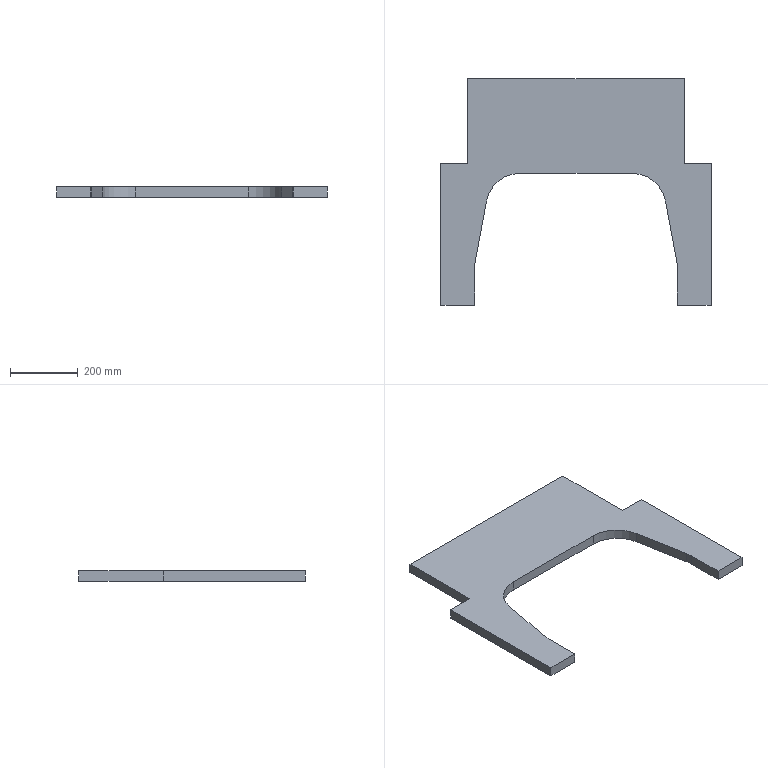Component | SolidWorks | JF21-80.1-1-3(_)-1-SOLID34-1 | 1 solid | 20 faces | box 800 x 670 x 30 mm | volume 8347939 mm3 | plane 16 | cylinder 4 | commonest cylinder face diameters 200 x4
STEP:
#1=COLOUR_RGB('',0.7922,0.8196,0.9333);
#2=FILL_AREA_STYLE_COLOUR('',#1);
#3=FILL_AREA_STYLE('',(#2));
#4=SURFACE_STYLE_FILL_AREA(#3);
#5=SURFACE_SIDE_STYLE('',(#4));
#6=SURFACE_STYLE_USAGE(.BOTH.,#5);
#7=PRESENTATION_STYLE_ASSIGNMENT((#6));
#8=CARTESIAN_POINT('',(15.748,-72.047,7.677));
#9=VERTEX_POINT('',#8);
#10=CARTESIAN_POINT('',(12.598,-72.047,7.677));
#11=VERTEX_POINT('',#10);
#12=CARTESIAN_POINT('',(12.598,-72.047,7.677));
#13=DIRECTION('',(-1.,0.,0.));
#14=VECTOR('',#13,39.37);
#15=LINE('',#12,#14);
#16=EDGE_CURVE('',#9,#11,#15,.T.);
#17=ORIENTED_EDGE('',*,*,#16,.T.);
#18=CARTESIAN_POINT('',(12.598,-72.047,8.858));
#19=VERTEX_POINT('',#18);
#20=CARTESIAN_POINT('',(12.598,-72.047,8.858));
#21=DIRECTION('',(0.,0.,-1.));
#22=VECTOR('',#21,39.37);
#23=LINE('',#20,#22);
#24=EDGE_CURVE('',#19,#11,#23,.T.);
#25=ORIENTED_EDGE('',*,*,#24,.F.);
#26=CARTESIAN_POINT('',(15.748,-72.047,8.858));
#27=VERTEX_POINT('',#26);
#28=CARTESIAN_POINT('',(12.598,-72.047,8.858));
#29=DIRECTION('',(-1.,0.,0.));
#30=VECTOR('',#29,39.37);
#31=LINE('',#28,#30);
#32=EDGE_CURVE('',#27,#19,#31,.T.);
#33=ORIENTED_EDGE('',*,*,#32,.F.);
#34=CARTESIAN_POINT('',(15.748,-72.047,8.858));
#35=DIRECTION('',(0.,0.,-1.));
#36=VECTOR('',#35,39.37);
#37=LINE('',#34,#36);
#38=EDGE_CURVE('',#27,#9,#37,.T.);
#39=ORIENTED_EDGE('',*,*,#38,.T.);
#40=EDGE_LOOP('',(#17,#25,#33,#39));
#41=FACE_OUTER_BOUND('',#40,.T.);
#42=CARTESIAN_POINT('',(12.598,-72.047,8.858));
#43=DIRECTION('',(0.,-1.,0.));
#44=DIRECTION('',(0.,0.,1.));
#45=AXIS2_PLACEMENT_3D('',#42,#43,#44);
#46=PLANE('',#45);
#47=ADVANCED_FACE('',(#41),#46,.F.);
#48=CARTESIAN_POINT('',(12.598,-62.205,7.677));
#49=VERTEX_POINT('',#48);
#50=CARTESIAN_POINT('',(12.598,-72.047,7.677));
#51=DIRECTION('',(0.,1.,0.));
#52=VECTOR('',#51,39.37);
#53=LINE('',#50,#52);
#54=EDGE_CURVE('',#11,#49,#53,.T.);
#55=ORIENTED_EDGE('',*,*,#54,.T.);
#56=CARTESIAN_POINT('',(12.598,-62.205,8.858));
#57=VERTEX_POINT('',#56);
#58=CARTESIAN_POINT('',(12.598,-62.205,8.858));
#59=DIRECTION('',(0.,0.,-1.));
#60=VECTOR('',#59,39.37);
#61=LINE('',#58,#60);
#62=EDGE_CURVE('',#57,#49,#61,.T.);
#63=ORIENTED_EDGE('',*,*,#62,.F.);
#64=CARTESIAN_POINT('',(12.598,-72.047,8.858));
#65=DIRECTION('',(0.,1.,0.));
#66=VECTOR('',#65,39.37);
#67=LINE('',#64,#66);
#68=EDGE_CURVE('',#19,#57,#67,.T.);
#69=ORIENTED_EDGE('',*,*,#68,.F.);
#70=ORIENTED_EDGE('',*,*,#24,.T.);
#71=EDGE_LOOP('',(#55,#63,#69,#70));
#72=FACE_OUTER_BOUND('',#71,.T.);
#73=CARTESIAN_POINT('',(12.598,-72.047,8.858));
#74=DIRECTION('',(-1.,0.,0.));
#75=DIRECTION('',(0.,0.,-1.));
#76=AXIS2_PLACEMENT_3D('',#73,#74,#75);
#77=PLANE('',#76);
#78=ADVANCED_FACE('',(#72),#77,.F.);
#79=CARTESIAN_POINT('',(-12.598,-62.205,7.677));
#80=VERTEX_POINT('',#79);
#81=CARTESIAN_POINT('',(-12.598,-62.205,7.677));
#82=DIRECTION('',(-1.,0.,0.));
#83=VECTOR('',#82,39.37);
#84=LINE('',#81,#83);
#85=EDGE_CURVE('',#49,#80,#84,.T.);
#86=ORIENTED_EDGE('',*,*,#85,.T.);
#87=CARTESIAN_POINT('',(-12.598,-62.205,8.858));
#88=VERTEX_POINT('',#87);
#89=CARTESIAN_POINT('',(-12.598,-62.205,8.858));
#90=DIRECTION('',(0.,0.,-1.));
#91=VECTOR('',#90,39.37);
#92=LINE('',#89,#91);
#93=EDGE_CURVE('',#88,#80,#92,.T.);
#94=ORIENTED_EDGE('',*,*,#93,.F.);
#95=CARTESIAN_POINT('',(-12.598,-62.205,8.858));
#96=DIRECTION('',(-1.,0.,0.));
#97=VECTOR('',#96,39.37);
#98=LINE('',#95,#97);
#99=EDGE_CURVE('',#57,#88,#98,.T.);
#100=ORIENTED_EDGE('',*,*,#99,.F.);
#101=ORIENTED_EDGE('',*,*,#62,.T.);
#102=EDGE_LOOP('',(#86,#94,#100,#101));
#103=FACE_OUTER_BOUND('',#102,.T.);
#104=CARTESIAN_POINT('',(-12.598,-62.205,8.858));
#105=DIRECTION('',(0.,-1.,0.));
#106=DIRECTION('',(0.,0.,1.));
#107=AXIS2_PLACEMENT_3D('',#104,#105,#106);
#108=PLANE('',#107);
#109=ADVANCED_FACE('',(#103),#108,.F.);
#110=CARTESIAN_POINT('',(-12.598,-72.047,7.677));
#111=VERTEX_POINT('',#110);
#112=CARTESIAN_POINT('',(-12.598,-72.047,7.677));
#113=DIRECTION('',(0.,-1.,0.));
#114=VECTOR('',#113,39.37);
#115=LINE('',#112,#114);
#116=EDGE_CURVE('',#80,#111,#115,.T.);
#117=ORIENTED_EDGE('',*,*,#116,.T.);
#118=CARTESIAN_POINT('',(-12.598,-72.047,8.858));
#119=VERTEX_POINT('',#118);
#120=CARTESIAN_POINT('',(-12.598,-72.047,8.858));
#121=DIRECTION('',(0.,0.,-1.));
#122=VECTOR('',#121,39.37);
#123=LINE('',#120,#122);
#124=EDGE_CURVE('',#119,#111,#123,.T.);
#125=ORIENTED_EDGE('',*,*,#124,.F.);
#126=CARTESIAN_POINT('',(-12.598,-72.047,8.858));
#127=DIRECTION('',(0.,-1.,0.));
#128=VECTOR('',#127,39.37);
#129=LINE('',#126,#128);
#130=EDGE_CURVE('',#88,#119,#129,.T.);
#131=ORIENTED_EDGE('',*,*,#130,.F.);
#132=ORIENTED_EDGE('',*,*,#93,.T.);
#133=EDGE_LOOP('',(#117,#125,#131,#132));
#134=FACE_OUTER_BOUND('',#133,.T.);
#135=CARTESIAN_POINT('',(-12.598,-72.047,8.858));
#136=DIRECTION('',(1.,0.,0.));
#137=DIRECTION('',(0.,0.,1.));
#138=AXIS2_PLACEMENT_3D('',#135,#136,#137);
#139=PLANE('',#138);
#140=ADVANCED_FACE('',(#134),#139,.F.);
#141=CARTESIAN_POINT('',(-15.748,-72.047,7.677));
#142=VERTEX_POINT('',#141);
#143=CARTESIAN_POINT('',(-12.598,-72.047,7.677));
#144=DIRECTION('',(-1.,0.,0.));
#145=VECTOR('',#144,39.37);
#146=LINE('',#143,#145);
#147=EDGE_CURVE('',#111,#142,#146,.T.);
#148=ORIENTED_EDGE('',*,*,#147,.T.);
#149=CARTESIAN_POINT('',(-15.748,-72.047,8.858));
#150=VERTEX_POINT('',#149);
#151=CARTESIAN_POINT('',(-15.748,-72.047,8.858));
#152=DIRECTION('',(0.,0.,-1.));
#153=VECTOR('',#152,39.37);
#154=LINE('',#151,#153);
#155=EDGE_CURVE('',#150,#142,#154,.T.);
#156=ORIENTED_EDGE('',*,*,#155,.F.);
#157=CARTESIAN_POINT('',(-12.598,-72.047,8.858));
#158=DIRECTION('',(-1.,0.,0.));
#159=VECTOR('',#158,39.37);
#160=LINE('',#157,#159);
#161=EDGE_CURVE('',#119,#150,#160,.T.);
#162=ORIENTED_EDGE('',*,*,#161,.F.);
#163=ORIENTED_EDGE('',*,*,#124,.T.);
#164=EDGE_LOOP('',(#148,#156,#162,#163));
#165=FACE_OUTER_BOUND('',#164,.T.);
#166=CARTESIAN_POINT('',(-12.598,-72.047,8.858));
#167=DIRECTION('',(0.,-1.,0.));
#168=DIRECTION('',(0.,0.,1.));
#169=AXIS2_PLACEMENT_3D('',#166,#167,#168);
#170=PLANE('',#169);
#171=ADVANCED_FACE('',(#165),#170,.F.);
#172=CARTESIAN_POINT('',(-15.748,-88.583,7.677));
#173=VERTEX_POINT('',#172);
#174=CARTESIAN_POINT('',(-15.748,-72.047,7.677));
#175=DIRECTION('',(0.,-1.,0.));
#176=VECTOR('',#175,39.37);
#177=LINE('',#174,#176);
#178=EDGE_CURVE('',#142,#173,#177,.T.);
#179=ORIENTED_EDGE('',*,*,#178,.T.);
#180=CARTESIAN_POINT('',(-15.748,-88.583,8.858));
#181=VERTEX_POINT('',#180);
#182=CARTESIAN_POINT('',(-15.748,-88.583,8.858));
#183=DIRECTION('',(0.,0.,-1.));
#184=VECTOR('',#183,39.37);
#185=LINE('',#182,#184);
#186=EDGE_CURVE('',#181,#173,#185,.T.);
#187=ORIENTED_EDGE('',*,*,#186,.F.);
#188=CARTESIAN_POINT('',(-15.748,-72.047,8.858));
#189=DIRECTION('',(0.,-1.,0.));
#190=VECTOR('',#189,39.37);
#191=LINE('',#188,#190);
#192=EDGE_CURVE('',#150,#181,#191,.T.);
#193=ORIENTED_EDGE('',*,*,#192,.F.);
#194=ORIENTED_EDGE('',*,*,#155,.T.);
#195=EDGE_LOOP('',(#179,#187,#193,#194));
#196=FACE_OUTER_BOUND('',#195,.T.);
#197=CARTESIAN_POINT('',(-15.748,-72.047,8.858));
#198=DIRECTION('',(1.,0.,0.));
#199=DIRECTION('',(0.,0.,1.));
#200=AXIS2_PLACEMENT_3D('',#197,#198,#199);
#201=PLANE('',#200);
#202=ADVANCED_FACE('',(#196),#201,.F.);
#203=CARTESIAN_POINT('',(-11.811,-88.583,7.677));
#204=VERTEX_POINT('',#203);
#205=CARTESIAN_POINT('',(-11.811,-88.583,7.677));
#206=DIRECTION('',(1.,0.,0.));
#207=VECTOR('',#206,39.37);
#208=LINE('',#205,#207);
#209=EDGE_CURVE('',#173,#204,#208,.T.);
#210=ORIENTED_EDGE('',*,*,#209,.T.);
#211=CARTESIAN_POINT('',(-11.811,-88.583,8.858));
#212=VERTEX_POINT('',#211);
#213=CARTESIAN_POINT('',(-11.811,-88.583,8.858));
#214=DIRECTION('',(0.,0.,-1.));
#215=VECTOR('',#214,39.37);
#216=LINE('',#213,#215);
#217=EDGE_CURVE('',#212,#204,#216,.T.);
#218=ORIENTED_EDGE('',*,*,#217,.F.);
#219=CARTESIAN_POINT('',(-11.811,-88.583,8.858));
#220=DIRECTION('',(1.,0.,0.));
#221=VECTOR('',#220,39.37);
#222=LINE('',#219,#221);
#223=EDGE_CURVE('',#181,#212,#222,.T.);
#224=ORIENTED_EDGE('',*,*,#223,.F.);
#225=ORIENTED_EDGE('',*,*,#186,.T.);
#226=EDGE_LOOP('',(#210,#218,#224,#225));
#227=FACE_OUTER_BOUND('',#226,.T.);
#228=CARTESIAN_POINT('',(-11.811,-88.583,8.858));
#229=DIRECTION('',(0.,1.,0.));
#230=DIRECTION('',(0.,0.,-1.));
#231=AXIS2_PLACEMENT_3D('',#228,#229,#230);
#232=PLANE('',#231);
#233=ADVANCED_FACE('',(#227),#232,.F.);
#234=CARTESIAN_POINT('',(-11.811,-84.22,7.677));
#235=VERTEX_POINT('',#234);
#236=CARTESIAN_POINT('',(-11.811,-84.22,7.677));
#237=DIRECTION('',(0.,1.,0.));
#238=VECTOR('',#237,39.37);
#239=LINE('',#236,#238);
#240=EDGE_CURVE('',#204,#235,#239,.T.);
#241=ORIENTED_EDGE('',*,*,#240,.T.);
#242=CARTESIAN_POINT('',(-11.811,-84.22,8.858));
#243=VERTEX_POINT('',#242);
#244=CARTESIAN_POINT('',(-11.811,-84.22,8.858));
#245=DIRECTION('',(0.,0.,-1.));
#246=VECTOR('',#245,39.37);
#247=LINE('',#244,#246);
#248=EDGE_CURVE('',#243,#235,#247,.T.);
#249=ORIENTED_EDGE('',*,*,#248,.F.);
#250=CARTESIAN_POINT('',(-11.811,-84.22,8.858));
#251=DIRECTION('',(0.,1.,0.));
#252=VECTOR('',#251,39.37);
#253=LINE('',#250,#252);
#254=EDGE_CURVE('',#212,#243,#253,.T.);
#255=ORIENTED_EDGE('',*,*,#254,.F.);
#256=ORIENTED_EDGE('',*,*,#217,.T.);
#257=EDGE_LOOP('',(#241,#249,#255,#256));
#258=FACE_OUTER_BOUND('',#257,.T.);
#259=CARTESIAN_POINT('',(-11.811,-84.22,8.858));
#260=DIRECTION('',(-1.,0.,0.));
#261=DIRECTION('',(0.,0.,-1.));
#262=AXIS2_PLACEMENT_3D('',#259,#260,#261);
#263=PLANE('',#262);
#264=ADVANCED_FACE('',(#258),#263,.F.);
#265=CARTESIAN_POINT('',(-11.745,-83.503,7.677));
#266=VERTEX_POINT('',#265);
#267=CARTESIAN_POINT('',(-7.874,-84.22,7.677));
#268=DIRECTION('',(0.,0.,-1.));
#269=DIRECTION('',(1.,0.,0.));
#270=AXIS2_PLACEMENT_3D('',#267,#268,#269);
#271=CIRCLE('',#270,3.937);
#272=EDGE_CURVE('',#235,#266,#271,.T.);
#273=ORIENTED_EDGE('',*,*,#272,.T.);
#274=CARTESIAN_POINT('',(-11.745,-83.503,8.858));
#275=VERTEX_POINT('',#274);
#276=CARTESIAN_POINT('',(-11.745,-83.503,8.858));
#277=DIRECTION('',(0.,0.,-1.));
#278=VECTOR('',#277,39.37);
#279=LINE('',#276,#278);
#280=EDGE_CURVE('',#275,#266,#279,.T.);
#281=ORIENTED_EDGE('',*,*,#280,.F.);
#282=CARTESIAN_POINT('',(-7.874,-84.22,8.858));
#283=DIRECTION('',(0.,0.,-1.));
#284=DIRECTION('',(1.,0.,0.));
#285=AXIS2_PLACEMENT_3D('',#282,#283,#284);
#286=CIRCLE('',#285,3.937);
#287=EDGE_CURVE('',#243,#275,#286,.T.);
#288=ORIENTED_EDGE('',*,*,#287,.F.);
#289=ORIENTED_EDGE('',*,*,#248,.T.);
#290=EDGE_LOOP('',(#273,#281,#288,#289));
#291=FACE_OUTER_BOUND('',#290,.T.);
#292=CARTESIAN_POINT('',(-7.874,-84.22,8.858));
#293=DIRECTION('',(0.,0.,-1.));
#294=DIRECTION('',(1.,0.,0.));
#295=AXIS2_PLACEMENT_3D('',#292,#293,#294);
#296=CYLINDRICAL_SURFACE('',#295,3.937);
#297=ADVANCED_FACE('',(#291),#296,.F.);
#298=CARTESIAN_POINT('',(-10.439,-76.448,7.677));
#299=VERTEX_POINT('',#298);
#300=CARTESIAN_POINT('',(-10.439,-76.448,7.677));
#301=DIRECTION('',(0.1821,0.9833,0.));
#302=VECTOR('',#301,39.37);
#303=LINE('',#300,#302);
#304=EDGE_CURVE('',#266,#299,#303,.T.);
#305=ORIENTED_EDGE('',*,*,#304,.T.);
#306=CARTESIAN_POINT('',(-10.439,-76.448,8.858));
#307=VERTEX_POINT('',#306);
#308=CARTESIAN_POINT('',(-10.439,-76.448,8.858));
#309=DIRECTION('',(0.,0.,-1.));
#310=VECTOR('',#309,39.37);
#311=LINE('',#308,#310);
#312=EDGE_CURVE('',#307,#299,#311,.T.);
#313=ORIENTED_EDGE('',*,*,#312,.F.);
#314=CARTESIAN_POINT('',(-10.439,-76.448,8.858));
#315=DIRECTION('',(0.1821,0.9833,0.));
#316=VECTOR('',#315,39.37);
#317=LINE('',#314,#316);
#318=EDGE_CURVE('',#275,#307,#317,.T.);
#319=ORIENTED_EDGE('',*,*,#318,.F.);
#320=ORIENTED_EDGE('',*,*,#280,.T.);
#321=EDGE_LOOP('',(#305,#313,#319,#320));
#322=FACE_OUTER_BOUND('',#321,.T.);
#323=CARTESIAN_POINT('',(-10.439,-76.448,8.858));
#324=DIRECTION('',(-0.9833,0.1821,0.));
#325=DIRECTION('',(0.1821,0.9833,0.));
#326=AXIS2_PLACEMENT_3D('',#323,#324,#325);
#327=PLANE('',#326);
#328=ADVANCED_FACE('',(#322),#327,.F.);
#329=CARTESIAN_POINT('',(-6.568,-73.228,7.677));
#330=VERTEX_POINT('',#329);
#331=CARTESIAN_POINT('',(-6.568,-77.165,7.677));
#332=DIRECTION('',(0.,0.,-1.));
#333=DIRECTION('',(1.,0.,0.));
#334=AXIS2_PLACEMENT_3D('',#331,#332,#333);
#335=CIRCLE('',#334,3.937);
#336=EDGE_CURVE('',#299,#330,#335,.T.);
#337=ORIENTED_EDGE('',*,*,#336,.T.);
#338=CARTESIAN_POINT('',(-6.568,-73.228,8.858));
#339=VERTEX_POINT('',#338);
#340=CARTESIAN_POINT('',(-6.568,-73.228,8.858));
#341=DIRECTION('',(0.,0.,-1.));
#342=VECTOR('',#341,39.37);
#343=LINE('',#340,#342);
#344=EDGE_CURVE('',#339,#330,#343,.T.);
#345=ORIENTED_EDGE('',*,*,#344,.F.);
#346=CARTESIAN_POINT('',(-6.568,-77.165,8.858));
#347=DIRECTION('',(0.,0.,-1.));
#348=DIRECTION('',(1.,0.,0.));
#349=AXIS2_PLACEMENT_3D('',#346,#347,#348);
#350=CIRCLE('',#349,3.937);
#351=EDGE_CURVE('',#307,#339,#350,.T.);
#352=ORIENTED_EDGE('',*,*,#351,.F.);
#353=ORIENTED_EDGE('',*,*,#312,.T.);
#354=EDGE_LOOP('',(#337,#345,#352,#353));
#355=FACE_OUTER_BOUND('',#354,.T.);
#356=CARTESIAN_POINT('',(-6.568,-77.165,8.858));
#357=DIRECTION('',(0.,0.,-1.));
#358=DIRECTION('',(1.,0.,0.));
#359=AXIS2_PLACEMENT_3D('',#356,#357,#358);
#360=CYLINDRICAL_SURFACE('',#359,3.937);
#361=ADVANCED_FACE('',(#355),#360,.F.);
#362=CARTESIAN_POINT('',(6.568,-73.228,7.677));
#363=VERTEX_POINT('',#362);
#364=CARTESIAN_POINT('',(6.568,-73.228,7.677));
#365=DIRECTION('',(1.,0.,0.));
#366=VECTOR('',#365,39.37);
#367=LINE('',#364,#366);
#368=EDGE_CURVE('',#330,#363,#367,.T.);
#369=ORIENTED_EDGE('',*,*,#368,.T.);
#370=CARTESIAN_POINT('',(6.568,-73.228,8.858));
#371=VERTEX_POINT('',#370);
#372=CARTESIAN_POINT('',(6.568,-73.228,8.858));
#373=DIRECTION('',(0.,0.,-1.));
#374=VECTOR('',#373,39.37);
#375=LINE('',#372,#374);
#376=EDGE_CURVE('',#371,#363,#375,.T.);
#377=ORIENTED_EDGE('',*,*,#376,.F.);
#378=CARTESIAN_POINT('',(6.568,-73.228,8.858));
#379=DIRECTION('',(1.,0.,0.));
#380=VECTOR('',#379,39.37);
#381=LINE('',#378,#380);
#382=EDGE_CURVE('',#339,#371,#381,.T.);
#383=ORIENTED_EDGE('',*,*,#382,.F.);
#384=ORIENTED_EDGE('',*,*,#344,.T.);
#385=EDGE_LOOP('',(#369,#377,#383,#384));
#386=FACE_OUTER_BOUND('',#385,.T.);
#387=CARTESIAN_POINT('',(6.568,-73.228,8.858));
#388=DIRECTION('',(0.,1.,0.));
#389=DIRECTION('',(0.,0.,-1.));
#390=AXIS2_PLACEMENT_3D('',#387,#388,#389);
#391=PLANE('',#390);
#392=ADVANCED_FACE('',(#386),#391,.F.);
#393=CARTESIAN_POINT('',(10.439,-76.448,7.677));
#394=VERTEX_POINT('',#393);
#395=CARTESIAN_POINT('',(6.568,-77.165,7.677));
#396=DIRECTION('',(0.,0.,-1.));
#397=DIRECTION('',(1.,0.,0.));
#398=AXIS2_PLACEMENT_3D('',#395,#396,#397);
#399=CIRCLE('',#398,3.937);
#400=EDGE_CURVE('',#363,#394,#399,.T.);
#401=ORIENTED_EDGE('',*,*,#400,.T.);
#402=CARTESIAN_POINT('',(10.439,-76.448,8.858));
#403=VERTEX_POINT('',#402);
#404=CARTESIAN_POINT('',(10.439,-76.448,8.858));
#405=DIRECTION('',(0.,0.,-1.));
#406=VECTOR('',#405,39.37);
#407=LINE('',#404,#406);
#408=EDGE_CURVE('',#403,#394,#407,.T.);
#409=ORIENTED_EDGE('',*,*,#408,.F.);
#410=CARTESIAN_POINT('',(6.568,-77.165,8.858));
#411=DIRECTION('',(0.,0.,-1.));
#412=DIRECTION('',(1.,0.,0.));
#413=AXIS2_PLACEMENT_3D('',#410,#411,#412);
#414=CIRCLE('',#413,3.937);
#415=EDGE_CURVE('',#371,#403,#414,.T.);
#416=ORIENTED_EDGE('',*,*,#415,.F.);
#417=ORIENTED_EDGE('',*,*,#376,.T.);
#418=EDGE_LOOP('',(#401,#409,#416,#417));
#419=FACE_OUTER_BOUND('',#418,.T.);
#420=CARTESIAN_POINT('',(6.568,-77.165,8.858));
#421=DIRECTION('',(0.,0.,-1.));
#422=DIRECTION('',(1.,0.,0.));
#423=AXIS2_PLACEMENT_3D('',#420,#421,#422);
#424=CYLINDRICAL_SURFACE('',#423,3.937);
#425=ADVANCED_FACE('',(#419),#424,.F.);
#426=CARTESIAN_POINT('',(11.745,-83.503,7.677));
#427=VERTEX_POINT('',#426);
#428=CARTESIAN_POINT('',(11.745,-83.503,7.677));
#429=DIRECTION('',(0.1821,-0.9833,0.));
#430=VECTOR('',#429,39.37);
#431=LINE('',#428,#430);
#432=EDGE_CURVE('',#394,#427,#431,.T.);
#433=ORIENTED_EDGE('',*,*,#432,.T.);
#434=CARTESIAN_POINT('',(11.745,-83.503,8.858));
#435=VERTEX_POINT('',#434);
#436=CARTESIAN_POINT('',(11.745,-83.503,8.858));
#437=DIRECTION('',(0.,0.,-1.));
#438=VECTOR('',#437,39.37);
#439=LINE('',#436,#438);
#440=EDGE_CURVE('',#435,#427,#439,.T.);
#441=ORIENTED_EDGE('',*,*,#440,.F.);
#442=CARTESIAN_POINT('',(11.745,-83.503,8.858));
#443=DIRECTION('',(0.1821,-0.9833,0.));
#444=VECTOR('',#443,39.37);
#445=LINE('',#442,#444);
#446=EDGE_CURVE('',#403,#435,#445,.T.);
#447=ORIENTED_EDGE('',*,*,#446,.F.);
#448=ORIENTED_EDGE('',*,*,#408,.T.);
#449=EDGE_LOOP('',(#433,#441,#447,#448));
#450=FACE_OUTER_BOUND('',#449,.T.);
#451=CARTESIAN_POINT('',(11.745,-83.503,8.858));
#452=DIRECTION('',(0.9833,0.1821,0.));
#453=DIRECTION('',(0.1821,-0.9833,0.));
#454=AXIS2_PLACEMENT_3D('',#451,#452,#453);
#455=PLANE('',#454);
#456=ADVANCED_FACE('',(#450),#455,.F.);
#457=CARTESIAN_POINT('',(11.811,-84.22,7.677));
#458=VERTEX_POINT('',#457);
#459=CARTESIAN_POINT('',(7.874,-84.22,7.677));
#460=DIRECTION('',(0.,0.,-1.));
#461=DIRECTION('',(1.,0.,0.));
#462=AXIS2_PLACEMENT_3D('',#459,#460,#461);
#463=CIRCLE('',#462,3.937);
#464=EDGE_CURVE('',#427,#458,#463,.T.);
#465=ORIENTED_EDGE('',*,*,#464,.T.);
#466=CARTESIAN_POINT('',(11.811,-84.22,8.858));
#467=VERTEX_POINT('',#466);
#468=CARTESIAN_POINT('',(11.811,-84.22,8.858));
#469=DIRECTION('',(0.,0.,-1.));
#470=VECTOR('',#469,39.37);
#471=LINE('',#468,#470);
#472=EDGE_CURVE('',#467,#458,#471,.T.);
#473=ORIENTED_EDGE('',*,*,#472,.F.);
#474=CARTESIAN_POINT('',(7.874,-84.22,8.858));
#475=DIRECTION('',(0.,0.,-1.));
#476=DIRECTION('',(1.,0.,0.));
#477=AXIS2_PLACEMENT_3D('',#474,#475,#476);
#478=CIRCLE('',#477,3.937);
#479=EDGE_CURVE('',#435,#467,#478,.T.);
#480=ORIENTED_EDGE('',*,*,#479,.F.);
#481=ORIENTED_EDGE('',*,*,#440,.T.);
#482=EDGE_LOOP('',(#465,#473,#480,#481));
#483=FACE_OUTER_BOUND('',#482,.T.);
#484=CARTESIAN_POINT('',(7.874,-84.22,8.858));
#485=DIRECTION('',(0.,0.,-1.));
#486=DIRECTION('',(1.,0.,0.));
#487=AXIS2_PLACEMENT_3D('',#484,#485,#486);
#488=CYLINDRICAL_SURFACE('',#487,3.937);
#489=ADVANCED_FACE('',(#483),#488,.F.);
#490=CARTESIAN_POINT('',(11.811,-88.583,7.677));
#491=VERTEX_POINT('',#490);
#492=CARTESIAN_POINT('',(11.811,-88.583,7.677));
#493=DIRECTION('',(-0.,-1.,0.));
#494=VECTOR('',#493,39.37);
#495=LINE('',#492,#494);
#496=EDGE_CURVE('',#458,#491,#495,.T.);
#497=ORIENTED_EDGE('',*,*,#496,.T.);
#498=CARTESIAN_POINT('',(11.811,-88.583,8.858));
#499=VERTEX_POINT('',#498);
#500=CARTESIAN_POINT('',(11.811,-88.583,8.858));
#501=DIRECTION('',(0.,0.,-1.));
#502=VECTOR('',#501,39.37);
#503=LINE('',#500,#502);
#504=EDGE_CURVE('',#499,#491,#503,.T.);
#505=ORIENTED_EDGE('',*,*,#504,.F.);
#506=CARTESIAN_POINT('',(11.811,-88.583,8.858));
#507=DIRECTION('',(-0.,-1.,0.));
#508=VECTOR('',#507,39.37);
#509=LINE('',#506,#508);
#510=EDGE_CURVE('',#467,#499,#509,.T.);
#511=ORIENTED_EDGE('',*,*,#510,.F.);
#512=ORIENTED_EDGE('',*,*,#472,.T.);
#513=EDGE_LOOP('',(#497,#505,#511,#512));
#514=FACE_OUTER_BOUND('',#513,.T.);
#515=CARTESIAN_POINT('',(11.811,-88.583,8.858));
#516=DIRECTION('',(1.,-0.,0.));
#517=DIRECTION('',(-0.,-1.,0.));
#518=AXIS2_PLACEMENT_3D('',#515,#516,#517);
#519=PLANE('',#518);
#520=ADVANCED_FACE('',(#514),#519,.F.);
#521=CARTESIAN_POINT('',(15.748,-88.583,7.677));
#522=VERTEX_POINT('',#521);
#523=CARTESIAN_POINT('',(15.748,-88.583,7.677));
#524=DIRECTION('',(1.,0.,0.));
#525=VECTOR('',#524,39.37);
#526=LINE('',#523,#525);
#527=EDGE_CURVE('',#491,#522,#526,.T.);
#528=ORIENTED_EDGE('',*,*,#527,.T.);
#529=CARTESIAN_POINT('',(15.748,-88.583,8.858));
#530=VERTEX_POINT('',#529);
#531=CARTESIAN_POINT('',(15.748,-88.583,8.858));
#532=DIRECTION('',(0.,0.,-1.));
#533=VECTOR('',#532,39.37);
#534=LINE('',#531,#533);
#535=EDGE_CURVE('',#530,#522,#534,.T.);
#536=ORIENTED_EDGE('',*,*,#535,.F.);
#537=CARTESIAN_POINT('',(15.748,-88.583,8.858));
#538=DIRECTION('',(1.,0.,0.));
#539=VECTOR('',#538,39.37);
#540=LINE('',#537,#539);
#541=EDGE_CURVE('',#499,#530,#540,.T.);
#542=ORIENTED_EDGE('',*,*,#541,.F.);
#543=ORIENTED_EDGE('',*,*,#504,.T.);
#544=EDGE_LOOP('',(#528,#536,#542,#543));
#545=FACE_OUTER_BOUND('',#544,.T.);
#546=CARTESIAN_POINT('',(15.748,-88.583,8.858));
#547=DIRECTION('',(0.,1.,0.));
#548=DIRECTION('',(0.,0.,-1.));
#549=AXIS2_PLACEMENT_3D('',#546,#547,#548);
#550=PLANE('',#549);
#551=ADVANCED_FACE('',(#545),#550,.F.);
#552=CARTESIAN_POINT('',(15.748,-72.047,7.677));
#553=DIRECTION('',(0.,1.,0.));
#554=VECTOR('',#553,39.37);
#555=LINE('',#552,#554);
#556=EDGE_CURVE('',#522,#9,#555,.T.);
#557=ORIENTED_EDGE('',*,*,#556,.T.);
#558=ORIENTED_EDGE('',*,*,#38,.F.);
#559=CARTESIAN_POINT('',(15.748,-72.047,8.858));
#560=DIRECTION('',(0.,1.,0.));
#561=VECTOR('',#560,39.37);
#562=LINE('',#559,#561);
#563=EDGE_CURVE('',#530,#27,#562,.T.);
#564=ORIENTED_EDGE('',*,*,#563,.F.);
#565=ORIENTED_EDGE('',*,*,#535,.T.);
#566=EDGE_LOOP('',(#557,#558,#564,#565));
#567=FACE_OUTER_BOUND('',#566,.T.);
#568=CARTESIAN_POINT('',(15.748,-72.047,8.858));
#569=DIRECTION('',(-1.,0.,0.));
#570=DIRECTION('',(0.,0.,-1.));
#571=AXIS2_PLACEMENT_3D('',#568,#569,#570);
#572=PLANE('',#571);
#573=ADVANCED_FACE('',(#567),#572,.F.);
#574=ORIENTED_EDGE('',*,*,#32,.T.);
#575=ORIENTED_EDGE('',*,*,#68,.T.);
#576=ORIENTED_EDGE('',*,*,#99,.T.);
#577=ORIENTED_EDGE('',*,*,#130,.T.);
#578=ORIENTED_EDGE('',*,*,#161,.T.);
#579=ORIENTED_EDGE('',*,*,#192,.T.);
#580=ORIENTED_EDGE('',*,*,#223,.T.);
#581=ORIENTED_EDGE('',*,*,#254,.T.);
#582=ORIENTED_EDGE('',*,*,#287,.T.);
#583=ORIENTED_EDGE('',*,*,#318,.T.);
#584=ORIENTED_EDGE('',*,*,#351,.T.);
#585=ORIENTED_EDGE('',*,*,#382,.T.);
#586=ORIENTED_EDGE('',*,*,#415,.T.);
#587=ORIENTED_EDGE('',*,*,#446,.T.);
#588=ORIENTED_EDGE('',*,*,#479,.T.);
#589=ORIENTED_EDGE('',*,*,#510,.T.);
#590=ORIENTED_EDGE('',*,*,#541,.T.);
#591=ORIENTED_EDGE('',*,*,#563,.T.);
#592=EDGE_LOOP('',(#574,#575,#576,#577,#578,#579,#580,#581,#582,#583,#584,#585,#586,#587,#588,#589,#590,#591));
#593=FACE_OUTER_BOUND('',#592,.T.);
#594=CARTESIAN_POINT('',(7.874,-84.22,8.858));
#595=DIRECTION('',(0.,0.,1.));
#596=DIRECTION('',(-1.,0.,0.));
#597=AXIS2_PLACEMENT_3D('',#594,#595,#596);
#598=PLANE('',#597);
#599=ADVANCED_FACE('',(#593),#598,.T.);
#600=ORIENTED_EDGE('',*,*,#16,.F.);
#601=ORIENTED_EDGE('',*,*,#556,.F.);
#602=ORIENTED_EDGE('',*,*,#527,.F.);
#603=ORIENTED_EDGE('',*,*,#496,.F.);
#604=ORIENTED_EDGE('',*,*,#464,.F.);
#605=ORIENTED_EDGE('',*,*,#432,.F.);
#606=ORIENTED_EDGE('',*,*,#400,.F.);
#607=ORIENTED_EDGE('',*,*,#368,.F.);
#608=ORIENTED_EDGE('',*,*,#336,.F.);
#609=ORIENTED_EDGE('',*,*,#304,.F.);
#610=ORIENTED_EDGE('',*,*,#272,.F.);
#611=ORIENTED_EDGE('',*,*,#240,.F.);
#612=ORIENTED_EDGE('',*,*,#209,.F.);
#613=ORIENTED_EDGE('',*,*,#178,.F.);
#614=ORIENTED_EDGE('',*,*,#147,.F.);
#615=ORIENTED_EDGE('',*,*,#116,.F.);
#616=ORIENTED_EDGE('',*,*,#85,.F.);
#617=ORIENTED_EDGE('',*,*,#54,.F.);
#618=EDGE_LOOP('',(#600,#601,#602,#603,#604,#605,#606,#607,#608,#609,#610,#611,#612,#613,#614,#615,#616,#617));
#619=FACE_OUTER_BOUND('',#618,.T.);
#620=CARTESIAN_POINT('',(7.874,-84.22,7.677));
#621=DIRECTION('',(0.,0.,1.));
#622=DIRECTION('',(-1.,0.,0.));
#623=AXIS2_PLACEMENT_3D('',#620,#621,#622);
#624=PLANE('',#623);
#625=ADVANCED_FACE('',(#619),#624,.F.);
#626=CLOSED_SHELL('',(#47,#78,#109,#140,#171,#202,#233,#264,#297,#328,#361,#392,#425,#456,#489,#520,#551,#573,#599,#625));
#627=MANIFOLD_SOLID_BREP('',#626);
#628=STYLED_ITEM('',(#7),#627);
#629=PRESENTATION_LAYER_ASSIGNMENT('','',(#628));
#630=(LENGTH_UNIT()NAMED_UNIT(*)SI_UNIT($,.METRE.));
#631=LENGTH_MEASURE_WITH_UNIT(LENGTH_MEASURE(0.0254),#630);
#632=DIMENSIONAL_EXPONENTS(1.,0.,0.,0.,0.,0.,0.);
#633=(CONVERSION_BASED_UNIT('',#631)LENGTH_UNIT()NAMED_UNIT(#632));
#634=UNCERTAINTY_MEASURE_WITH_UNIT(LENGTH_MEASURE(0.00001),#633,'','');
#635=(NAMED_UNIT(*)PLANE_ANGLE_UNIT()SI_UNIT($,.RADIAN.));
#636=(NAMED_UNIT(*)SI_UNIT($,.STERADIAN.)SOLID_ANGLE_UNIT());
#637=(GEOMETRIC_REPRESENTATION_CONTEXT(3)GLOBAL_UNCERTAINTY_ASSIGNED_CONTEXT((#634))GLOBAL_UNIT_ASSIGNED_CONTEXT((#633,#635,#636))REPRESENTATION_CONTEXT('',''));
#638=MECHANICAL_DESIGN_GEOMETRIC_PRESENTATION_REPRESENTATION('',(#628),#637);
#639=CARTESIAN_POINT('',(0.,0.,0.));
#640=DIRECTION('',(0.,0.,1.));
#641=DIRECTION('',(1.,0.,0.));
#642=AXIS2_PLACEMENT_3D('',#639,#640,#641);
#643=(LENGTH_UNIT()NAMED_UNIT(*)SI_UNIT($,.METRE.));
#644=LENGTH_MEASURE_WITH_UNIT(LENGTH_MEASURE(0.0254),#643);
#645=DIMENSIONAL_EXPONENTS(1.,0.,0.,0.,0.,0.,0.);
#646=(CONVERSION_BASED_UNIT('',#644)LENGTH_UNIT()NAMED_UNIT(#645));
#647=UNCERTAINTY_MEASURE_WITH_UNIT(LENGTH_MEASURE(0.00001),#646,'','');
#648=(NAMED_UNIT(*)PLANE_ANGLE_UNIT()SI_UNIT($,.RADIAN.));
#649=(NAMED_UNIT(*)SI_UNIT($,.STERADIAN.)SOLID_ANGLE_UNIT());
#650=(GEOMETRIC_REPRESENTATION_CONTEXT(3)GLOBAL_UNCERTAINTY_ASSIGNED_CONTEXT((#647))GLOBAL_UNIT_ASSIGNED_CONTEXT((#646,#648,#649))REPRESENTATION_CONTEXT('',''));
#651=ADVANCED_BREP_SHAPE_REPRESENTATION('',(#627,#642),#650);